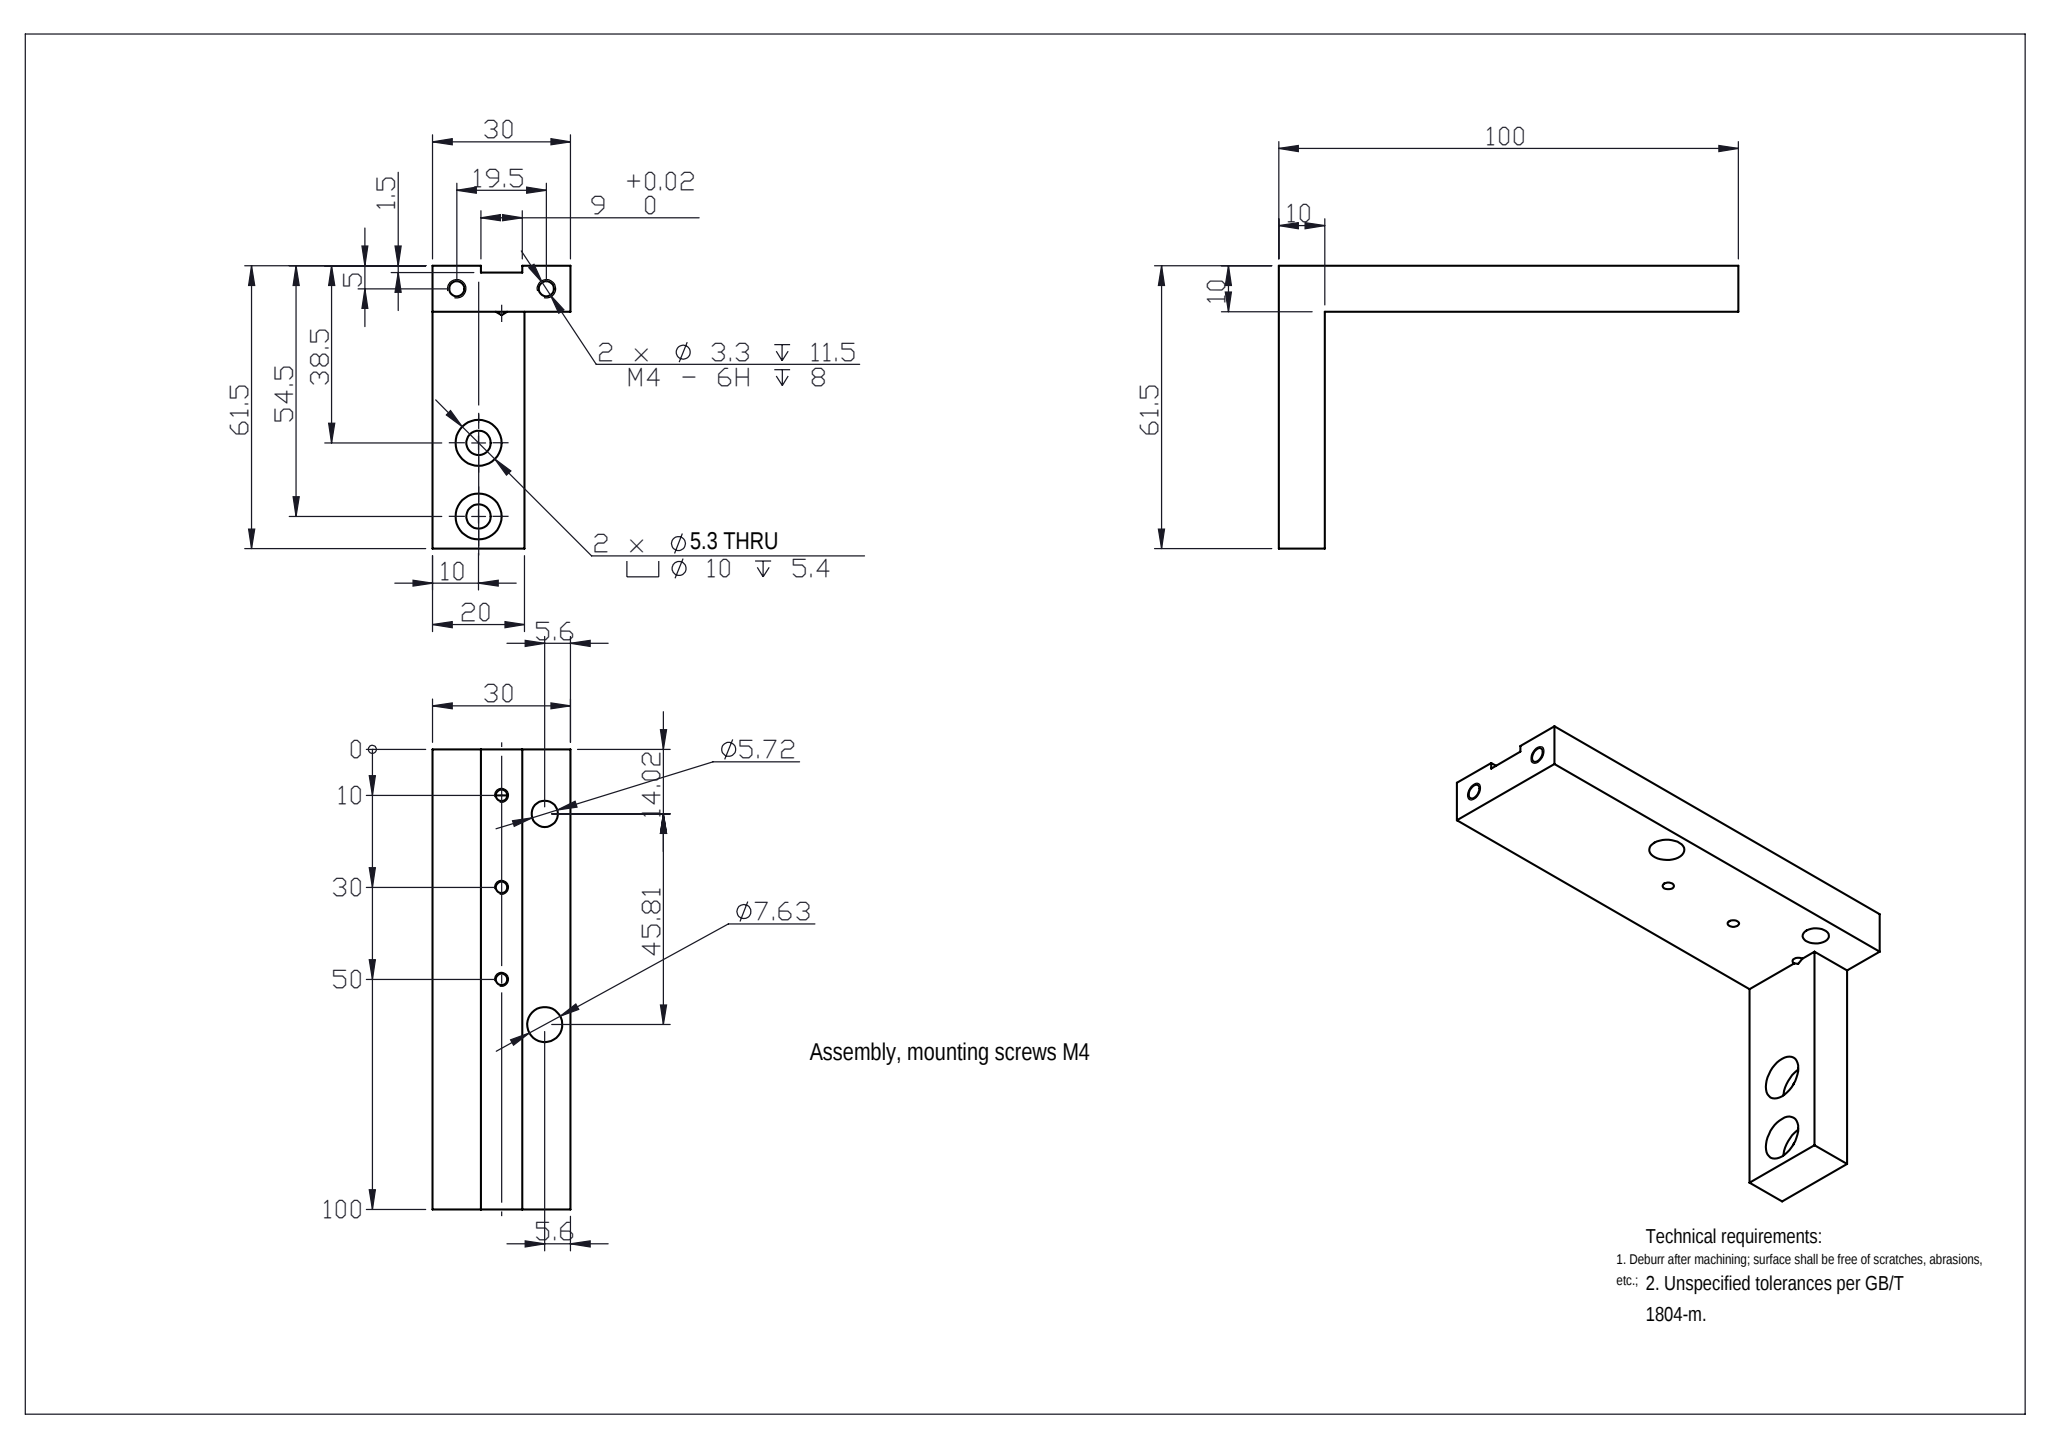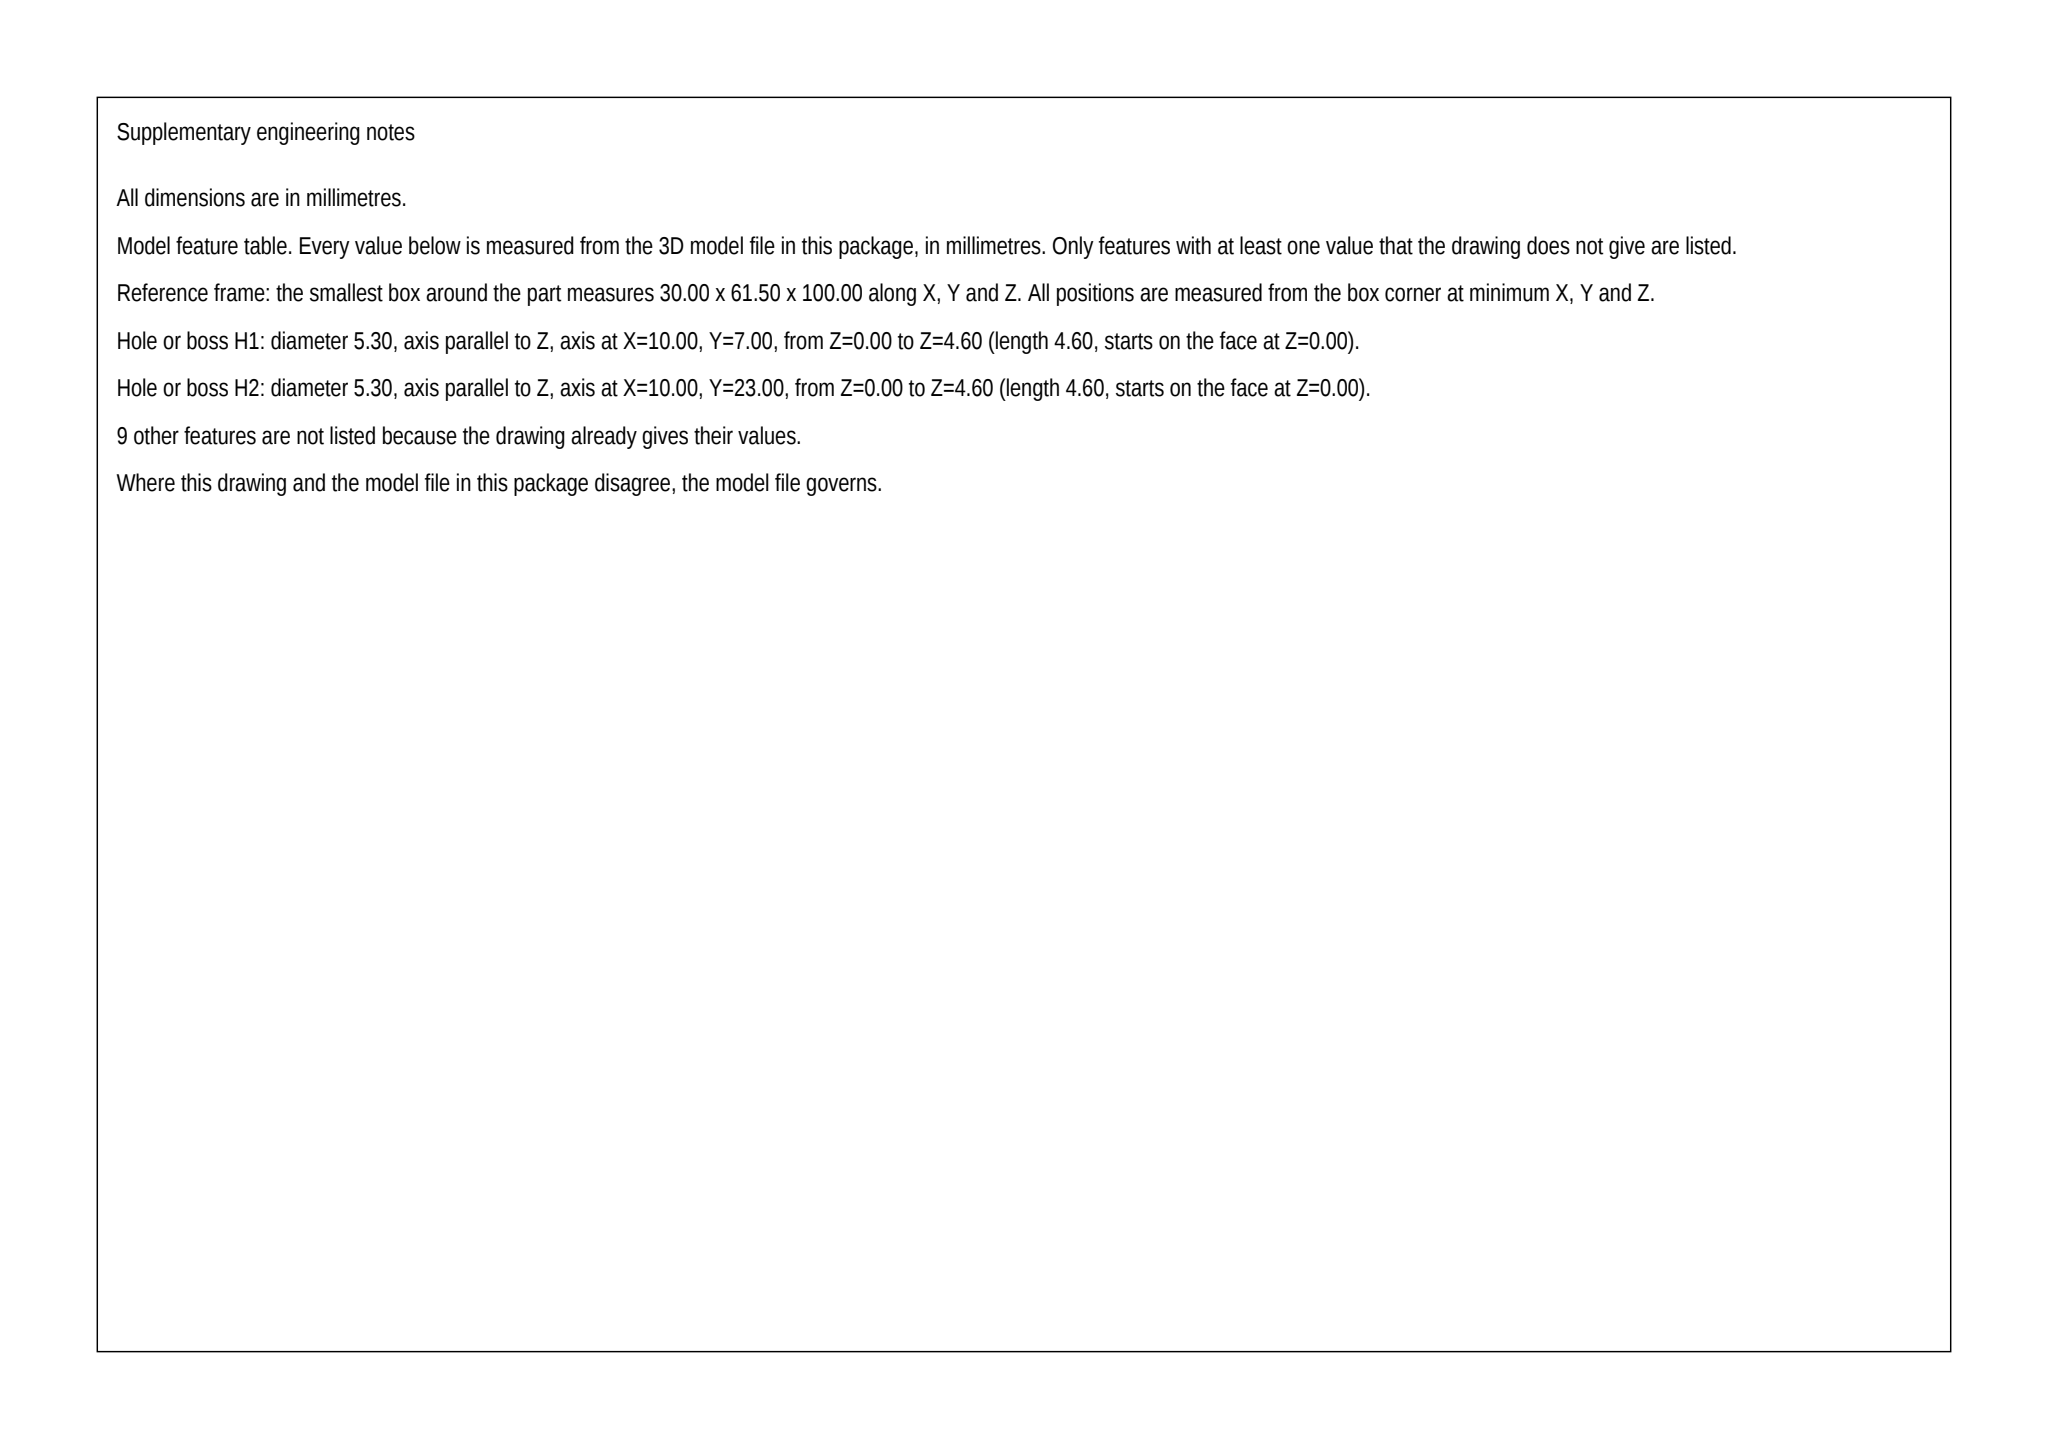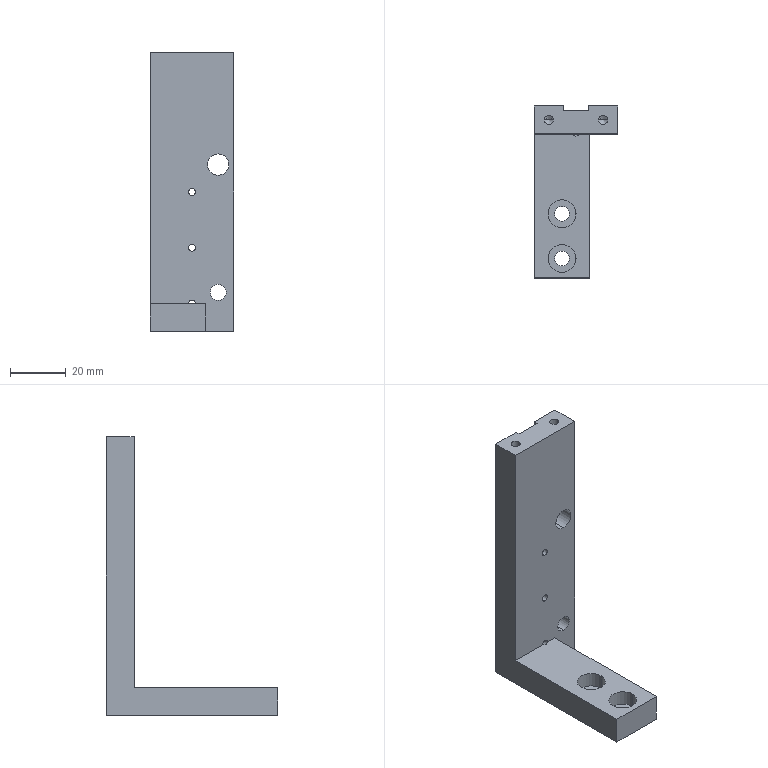Part | SolidWorks | mm | 1 solid | 42 faces | box 30 x 61.5 x 100 mm | volume 36856 mm3 | cylinder 22 | plane 15 | cone 5 | commonest cylinder face diameters 2.5 x6 3.3 x4 10 x4 5.3 x4 5.724 x2 7.634 x2
build123d program:
from build123d import *

# Parameters (mm, degrees)
SKETCH1_W                                       = 20
SKETCH1_H                                       = 51.5
BOSS_EXTRUDE1_DEPTH                             = 10
SKETCH2_W                                       = 30
SKETCH2_H                                       = 100
BOSS_EXTRUDE2_DEPTH                             = 10
M5_HEX_SOCKET_HEAD_CAP_SCREW_CBORE1_D           = 5.3
M5_HEX_SOCKET_HEAD_CAP_SCREW_CBORE1_CBORE_D     = 10
M5_HEX_SOCKET_HEAD_CAP_SCREW_CBORE1_CBORE_DEPTH = 5.4
SKETCH5_W                                       = 9
SKETCH5_H                                       = 100
CUT_EXTRUDE1_DEPTH                              = 1.5
M3_TAPPED_HOLE1_D                               = 2.5
M3_TAPPED_HOLE1_DEPTH                           = 8.5
M3_TAPPED_HOLE1_TIP                             = 0.7511
M4_TAPPED_HOLE1_D                               = 3.3
M4_TAPPED_HOLE1_DEPTH                           = 11.5
M4_TAPPED_HOLE1_TIP                             = 0.9914
SKETCH10_R                                      = 2.862
SKETCH10_R_2                                    = 3.817
CUT_EXTRUDE2_DEPTH                              = 15


with BuildPart() as part:
    # Sketch1 → Boss-Extrude1 (new body)
    with BuildSketch(Plane.XY):
        with Locations((10, -25.75)):
            Rectangle(SKETCH1_W, SKETCH1_H)
    extrude(amount=BOSS_EXTRUDE1_DEPTH)

    # Sketch2 → Boss-Extrude2 (add)
    with BuildSketch(Plane(origin=(0, 0, 0), x_dir=(1, 0, 0), z_dir=(0, 1, 0))):
        with Locations((15, -50)):
            Rectangle(SKETCH2_W, SKETCH2_H)
    extrude(amount=BOSS_EXTRUDE2_DEPTH)

    # M5 Hex Socket Head Cap Screw CBORE1 (through all)
    with Locations(Plane.XY.offset(10)):
        with Locations((10, -28.5), (10, -44.5)):
            CounterBoreHole(M5_HEX_SOCKET_HEAD_CAP_SCREW_CBORE1_D / 2, M5_HEX_SOCKET_HEAD_CAP_SCREW_CBORE1_CBORE_D / 2, M5_HEX_SOCKET_HEAD_CAP_SCREW_CBORE1_CBORE_DEPTH)

    # Sketch5 → Cut-Extrude1 (cut)
    with BuildSketch(Plane(origin=(0, 10, 0), x_dir=(1, 0, 0), z_dir=(0, 1, 0))):
        with Locations((15, -50)):
            Rectangle(SKETCH5_W, SKETCH5_H)
    extrude(amount=-CUT_EXTRUDE1_DEPTH, mode=Mode.SUBTRACT)

    # M3 Tapped Hole1
    with Locations(Plane(origin=(0, 8.5, 0), x_dir=(1, 0, 0), z_dir=(0, 1, 0))):
        with Locations((15, -10), (15, -30), (15, -50)):
            Hole(M3_TAPPED_HOLE1_D / 2, depth=M3_TAPPED_HOLE1_DEPTH)
            with Locations((0, 0, -(M3_TAPPED_HOLE1_DEPTH + M3_TAPPED_HOLE1_TIP / 2))):  # 118° drill point
                Cone(0, M3_TAPPED_HOLE1_D / 2, M3_TAPPED_HOLE1_TIP, mode=Mode.SUBTRACT)

    # M4 Tapped Hole1
    with Locations(Plane.XY.offset(100)):
        with Locations((5.25, 5), (24.75, 5)):
            Hole(M4_TAPPED_HOLE1_D / 2, depth=M4_TAPPED_HOLE1_DEPTH)
            with Locations((0, 0, -(M4_TAPPED_HOLE1_DEPTH + M4_TAPPED_HOLE1_TIP / 2))):  # 118° drill point
                Cone(0, M4_TAPPED_HOLE1_D / 2, M4_TAPPED_HOLE1_TIP, mode=Mode.SUBTRACT)

    # Sketch10 → Cut-Extrude2 (cut)
    with BuildSketch(Plane(origin=(0, 10, 0), x_dir=(1, 0, 0), z_dir=(0, 1, 0))):
        with Locations(Location((24.395, -14.017, 0), (0, 0, 270))):
            Circle(SKETCH10_R)
        with Locations(Location((24.395, -59.831, 0), (0, 0, 270))):
            Circle(SKETCH10_R_2)
    extrude(amount=-CUT_EXTRUDE2_DEPTH, mode=Mode.SUBTRACT)


solid = part.part